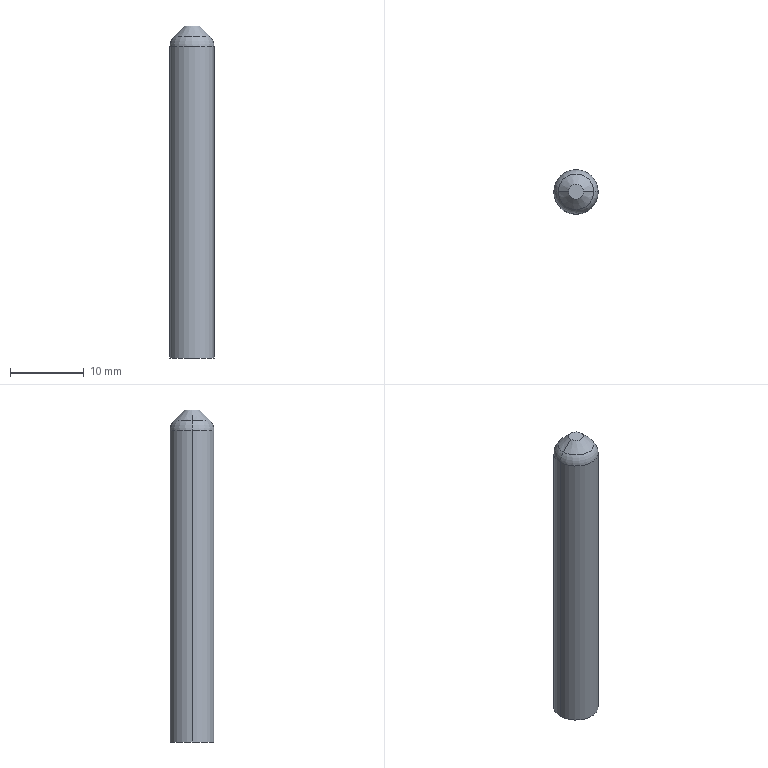Component | SolidWorks | Gripper-2024-3-4-08-1 | 1 solid | 8 faces | box 6 x 6 x 45 mm | volume 1241 mm3 | torus 2 | cone 2 | cylinder 2 | plane 2 | commonest cylinder face diameters 6 x2 | material S45C
build123d program:
from build123d import *

# Parameters (mm, degrees)
SKETCH1_R           = 3
BOSS_EXTRUDE1_DEPTH = 45
CHAMFER1_SIZE       = 2
FILLET1_R           = 2


with BuildPart() as part:
    # Sketch1 → Boss-Extrude1 (new body)
    with BuildSketch(Plane.XY):
        with Locations(Location((0, 0, 0), (0, 0, 180))):
            Circle(SKETCH1_R)
    extrude(amount=BOSS_EXTRUDE1_DEPTH)

    # Chamfer1
    chamfer1_edges = [part.edges().sort_by_distance(p)[0] for p in [
        (3, 0, 45),
    ]]
    chamfer(chamfer1_edges, length=CHAMFER1_SIZE)

    # Fillet1
    fillet1_edges = [part.edges().sort_by_distance(p)[0] for p in [
        (3, 0, 43),
    ]]
    fillet(fillet1_edges, radius=FILLET1_R)


solid = part.part

# Placed as in the assembly
solid = solid.moved(Location((-163.094, -123.769, 303), (0, 0, 0)))
STEP:
#1=COLOUR_RGB('',0.7922,0.8196,0.9333);
#2=FILL_AREA_STYLE_COLOUR('',#1);
#3=FILL_AREA_STYLE('',(#2));
#4=SURFACE_STYLE_FILL_AREA(#3);
#5=SURFACE_SIDE_STYLE('',(#4));
#6=SURFACE_STYLE_USAGE(.BOTH.,#5);
#7=PRESENTATION_STYLE_ASSIGNMENT((#6));
#8=CARTESIAN_POINT('',(-6.539,-4.873,13.589));
#9=VERTEX_POINT('',#8);
#10=CARTESIAN_POINT('',(-6.303,-4.873,13.589));
#11=VERTEX_POINT('',#10);
#12=CARTESIAN_POINT('',(-6.421,-4.873,13.589));
#13=DIRECTION('',(0.,0.,-1.));
#14=DIRECTION('',(1.,0.,0.));
#15=AXIS2_PLACEMENT_3D('',#12,#13,#14);
#16=CIRCLE('',#15,0.1181);
#17=EDGE_CURVE('',#9,#11,#16,.T.);
#18=ORIENTED_EDGE('',*,*,#17,.F.);
#19=CARTESIAN_POINT('',(-6.516,-4.873,13.645));
#20=VERTEX_POINT('',#19);
#21=CARTESIAN_POINT('',(-6.46,-4.873,13.589));
#22=DIRECTION('',(0.,1.,0.));
#23=DIRECTION('',(-1.,0.,0.));
#24=AXIS2_PLACEMENT_3D('',#21,#22,#23);
#25=CIRCLE('',#24,0.07874);
#26=EDGE_CURVE('',#9,#20,#25,.T.);
#27=ORIENTED_EDGE('',*,*,#26,.T.);
#28=CARTESIAN_POINT('',(-6.326,-4.873,13.645));
#29=VERTEX_POINT('',#28);
#30=CARTESIAN_POINT('',(-6.421,-4.873,13.645));
#31=DIRECTION('',(0.,0.,1.));
#32=DIRECTION('',(-1.,0.,0.));
#33=AXIS2_PLACEMENT_3D('',#30,#31,#32);
#34=CIRCLE('',#33,0.09505);
#35=EDGE_CURVE('',#29,#20,#34,.T.);
#36=ORIENTED_EDGE('',*,*,#35,.F.);
#37=CARTESIAN_POINT('',(-6.382,-4.873,13.589));
#38=DIRECTION('',(0.,-1.,0.));
#39=DIRECTION('',(0.,0.,-1.));
#40=AXIS2_PLACEMENT_3D('',#37,#38,#39);
#41=CIRCLE('',#40,0.07874);
#42=EDGE_CURVE('',#11,#29,#41,.T.);
#43=ORIENTED_EDGE('',*,*,#42,.F.);
#44=EDGE_LOOP('',(#18,#27,#36,#43));
#45=FACE_OUTER_BOUND('',#44,.T.);
#46=CARTESIAN_POINT('',(-6.421,-4.873,13.589));
#47=DIRECTION('',(0.,0.,1.));
#48=DIRECTION('',(1.,0.,0.));
#49=AXIS2_PLACEMENT_3D('',#46,#47,#48);
#50=TOROIDAL_SURFACE('',#49,0.03937,0.07874);
#51=ADVANCED_FACE('',(#45),#50,.T.);
#52=CARTESIAN_POINT('',(-6.382,-4.873,13.701));
#53=VERTEX_POINT('',#52);
#54=CARTESIAN_POINT('',(-6.46,-4.873,13.701));
#55=VERTEX_POINT('',#54);
#56=CARTESIAN_POINT('',(-6.421,-4.873,13.701));
#57=DIRECTION('',(0.,0.,1.));
#58=DIRECTION('',(1.,0.,0.));
#59=AXIS2_PLACEMENT_3D('',#56,#57,#58);
#60=CIRCLE('',#59,0.03937);
#61=EDGE_CURVE('',#53,#55,#60,.T.);
#62=ORIENTED_EDGE('',*,*,#61,.F.);
#63=CARTESIAN_POINT('',(-6.382,-4.873,13.701));
#64=DIRECTION('',(0.7071,0.,-0.7071));
#65=VECTOR('',#64,39.37);
#66=LINE('',#63,#65);
#67=EDGE_CURVE('',#53,#29,#66,.T.);
#68=ORIENTED_EDGE('',*,*,#67,.T.);
#69=ORIENTED_EDGE('',*,*,#35,.T.);
#70=CARTESIAN_POINT('',(-6.46,-4.873,13.701));
#71=DIRECTION('',(-0.7071,0.,-0.7071));
#72=VECTOR('',#71,39.37);
#73=LINE('',#70,#72);
#74=EDGE_CURVE('',#55,#20,#73,.T.);
#75=ORIENTED_EDGE('',*,*,#74,.F.);
#76=EDGE_LOOP('',(#62,#68,#69,#75));
#77=FACE_OUTER_BOUND('',#76,.T.);
#78=CARTESIAN_POINT('',(-6.421,-4.873,13.701));
#79=DIRECTION('',(0.,0.,-1.));
#80=DIRECTION('',(-1.,0.,0.));
#81=AXIS2_PLACEMENT_3D('',#78,#79,#80);
#82=CONICAL_SURFACE('',#81,0.03937,0.7854);
#83=ADVANCED_FACE('',(#77),#82,.T.);
#84=ORIENTED_EDGE('',*,*,#17,.T.);
#85=CARTESIAN_POINT('',(-6.303,-4.873,11.929));
#86=VERTEX_POINT('',#85);
#87=CARTESIAN_POINT('',(-6.303,-4.873,13.701));
#88=DIRECTION('',(0.,0.,-1.));
#89=VECTOR('',#88,39.37);
#90=LINE('',#87,#89);
#91=EDGE_CURVE('',#11,#86,#90,.T.);
#92=ORIENTED_EDGE('',*,*,#91,.T.);
#93=CARTESIAN_POINT('',(-6.539,-4.873,11.929));
#94=VERTEX_POINT('',#93);
#95=CARTESIAN_POINT('',(-6.421,-4.873,11.929));
#96=DIRECTION('',(0.,0.,1.));
#97=DIRECTION('',(1.,0.,0.));
#98=AXIS2_PLACEMENT_3D('',#95,#96,#97);
#99=CIRCLE('',#98,0.1181);
#100=EDGE_CURVE('',#86,#94,#99,.T.);
#101=ORIENTED_EDGE('',*,*,#100,.T.);
#102=CARTESIAN_POINT('',(-6.539,-4.873,13.701));
#103=DIRECTION('',(0.,0.,-1.));
#104=VECTOR('',#103,39.37);
#105=LINE('',#102,#104);
#106=EDGE_CURVE('',#9,#94,#105,.T.);
#107=ORIENTED_EDGE('',*,*,#106,.F.);
#108=EDGE_LOOP('',(#84,#92,#101,#107));
#109=FACE_OUTER_BOUND('',#108,.T.);
#110=CARTESIAN_POINT('',(-6.421,-4.873,13.701));
#111=DIRECTION('',(0.,0.,-1.));
#112=DIRECTION('',(-1.,0.,0.));
#113=AXIS2_PLACEMENT_3D('',#110,#111,#112);
#114=CYLINDRICAL_SURFACE('',#113,0.1181);
#115=ADVANCED_FACE('',(#109),#114,.T.);
#116=ORIENTED_EDGE('',*,*,#91,.F.);
#117=CARTESIAN_POINT('',(-6.421,-4.873,13.589));
#118=DIRECTION('',(0.,0.,-1.));
#119=DIRECTION('',(1.,0.,0.));
#120=AXIS2_PLACEMENT_3D('',#117,#118,#119);
#121=CIRCLE('',#120,0.1181);
#122=EDGE_CURVE('',#11,#9,#121,.T.);
#123=ORIENTED_EDGE('',*,*,#122,.T.);
#124=ORIENTED_EDGE('',*,*,#106,.T.);
#125=CARTESIAN_POINT('',(-6.421,-4.873,11.929));
#126=DIRECTION('',(0.,0.,1.));
#127=DIRECTION('',(1.,0.,0.));
#128=AXIS2_PLACEMENT_3D('',#125,#126,#127);
#129=CIRCLE('',#128,0.1181);
#130=EDGE_CURVE('',#94,#86,#129,.T.);
#131=ORIENTED_EDGE('',*,*,#130,.T.);
#132=EDGE_LOOP('',(#116,#123,#124,#131));
#133=FACE_OUTER_BOUND('',#132,.T.);
#134=CARTESIAN_POINT('',(-6.421,-4.873,13.701));
#135=DIRECTION('',(0.,0.,-1.));
#136=DIRECTION('',(-1.,0.,0.));
#137=AXIS2_PLACEMENT_3D('',#134,#135,#136);
#138=CYLINDRICAL_SURFACE('',#137,0.1181);
#139=ADVANCED_FACE('',(#133),#138,.T.);
#140=CARTESIAN_POINT('',(-6.421,-4.873,13.701));
#141=DIRECTION('',(0.,0.,1.));
#142=DIRECTION('',(1.,0.,0.));
#143=AXIS2_PLACEMENT_3D('',#140,#141,#142);
#144=CIRCLE('',#143,0.03937);
#145=EDGE_CURVE('',#55,#53,#144,.T.);
#146=ORIENTED_EDGE('',*,*,#145,.T.);
#147=ORIENTED_EDGE('',*,*,#61,.T.);
#148=EDGE_LOOP('',(#146,#147));
#149=FACE_OUTER_BOUND('',#148,.T.);
#150=CARTESIAN_POINT('',(-6.421,-4.873,13.701));
#151=DIRECTION('',(0.,0.,1.));
#152=DIRECTION('',(1.,0.,0.));
#153=AXIS2_PLACEMENT_3D('',#150,#151,#152);
#154=PLANE('',#153);
#155=ADVANCED_FACE('',(#149),#154,.T.);
#156=ORIENTED_EDGE('',*,*,#130,.F.);
#157=ORIENTED_EDGE('',*,*,#100,.F.);
#158=EDGE_LOOP('',(#156,#157));
#159=FACE_OUTER_BOUND('',#158,.T.);
#160=CARTESIAN_POINT('',(-6.421,-4.873,11.929));
#161=DIRECTION('',(0.,0.,1.));
#162=DIRECTION('',(1.,0.,0.));
#163=AXIS2_PLACEMENT_3D('',#160,#161,#162);
#164=PLANE('',#163);
#165=ADVANCED_FACE('',(#159),#164,.F.);
#166=ORIENTED_EDGE('',*,*,#67,.F.);
#167=ORIENTED_EDGE('',*,*,#145,.F.);
#168=ORIENTED_EDGE('',*,*,#74,.T.);
#169=CARTESIAN_POINT('',(-6.421,-4.873,13.645));
#170=DIRECTION('',(0.,0.,1.));
#171=DIRECTION('',(-1.,0.,0.));
#172=AXIS2_PLACEMENT_3D('',#169,#170,#171);
#173=CIRCLE('',#172,0.09505);
#174=EDGE_CURVE('',#20,#29,#173,.T.);
#175=ORIENTED_EDGE('',*,*,#174,.T.);
#176=EDGE_LOOP('',(#166,#167,#168,#175));
#177=FACE_OUTER_BOUND('',#176,.T.);
#178=CARTESIAN_POINT('',(-6.421,-4.873,13.701));
#179=DIRECTION('',(0.,0.,-1.));
#180=DIRECTION('',(-1.,0.,0.));
#181=AXIS2_PLACEMENT_3D('',#178,#179,#180);
#182=CONICAL_SURFACE('',#181,0.03937,0.7854);
#183=ADVANCED_FACE('',(#177),#182,.T.);
#184=ORIENTED_EDGE('',*,*,#26,.F.);
#185=ORIENTED_EDGE('',*,*,#122,.F.);
#186=ORIENTED_EDGE('',*,*,#42,.T.);
#187=ORIENTED_EDGE('',*,*,#174,.F.);
#188=EDGE_LOOP('',(#184,#185,#186,#187));
#189=FACE_OUTER_BOUND('',#188,.T.);
#190=CARTESIAN_POINT('',(-6.421,-4.873,13.589));
#191=DIRECTION('',(0.,0.,1.));
#192=DIRECTION('',(1.,0.,0.));
#193=AXIS2_PLACEMENT_3D('',#190,#191,#192);
#194=TOROIDAL_SURFACE('',#193,0.03937,0.07874);
#195=ADVANCED_FACE('',(#189),#194,.T.);
#196=CLOSED_SHELL('',(#51,#83,#115,#139,#155,#165,#183,#195));
#197=MANIFOLD_SOLID_BREP('',#196);
#198=STYLED_ITEM('',(#7),#197);
#199=(LENGTH_UNIT()NAMED_UNIT(*)SI_UNIT($,.METRE.));
#200=LENGTH_MEASURE_WITH_UNIT(LENGTH_MEASURE(0.0254),#199);
#201=DIMENSIONAL_EXPONENTS(1.,0.,0.,0.,0.,0.,0.);
#202=(CONVERSION_BASED_UNIT('',#200)LENGTH_UNIT()NAMED_UNIT(#201));
#203=UNCERTAINTY_MEASURE_WITH_UNIT(LENGTH_MEASURE(0.00001),#202,'','');
#204=(NAMED_UNIT(*)PLANE_ANGLE_UNIT()SI_UNIT($,.RADIAN.));
#205=(NAMED_UNIT(*)SI_UNIT($,.STERADIAN.)SOLID_ANGLE_UNIT());
#206=(GEOMETRIC_REPRESENTATION_CONTEXT(3)GLOBAL_UNCERTAINTY_ASSIGNED_CONTEXT((#203))GLOBAL_UNIT_ASSIGNED_CONTEXT((#202,#204,#205))REPRESENTATION_CONTEXT('',''));
#207=MECHANICAL_DESIGN_GEOMETRIC_PRESENTATION_REPRESENTATION('',(#198),#206);
#208=PRESENTATION_LAYER_ASSIGNMENT('','',(#198));
#209=CARTESIAN_POINT('',(0.,0.,0.));
#210=DIRECTION('',(0.,0.,1.));
#211=DIRECTION('',(1.,0.,0.));
#212=AXIS2_PLACEMENT_3D('',#209,#210,#211);
#213=(LENGTH_UNIT()NAMED_UNIT(*)SI_UNIT($,.METRE.));
#214=LENGTH_MEASURE_WITH_UNIT(LENGTH_MEASURE(0.0254),#213);
#215=DIMENSIONAL_EXPONENTS(1.,0.,0.,0.,0.,0.,0.);
#216=(CONVERSION_BASED_UNIT('',#214)LENGTH_UNIT()NAMED_UNIT(#215));
#217=UNCERTAINTY_MEASURE_WITH_UNIT(LENGTH_MEASURE(0.00001),#216,'','');
#218=(NAMED_UNIT(*)PLANE_ANGLE_UNIT()SI_UNIT($,.RADIAN.));
#219=(NAMED_UNIT(*)SI_UNIT($,.STERADIAN.)SOLID_ANGLE_UNIT());
#220=(GEOMETRIC_REPRESENTATION_CONTEXT(3)GLOBAL_UNCERTAINTY_ASSIGNED_CONTEXT((#217))GLOBAL_UNIT_ASSIGNED_CONTEXT((#216,#218,#219))REPRESENTATION_CONTEXT('',''));
#221=ADVANCED_BREP_SHAPE_REPRESENTATION('',(#197,#212),#220);